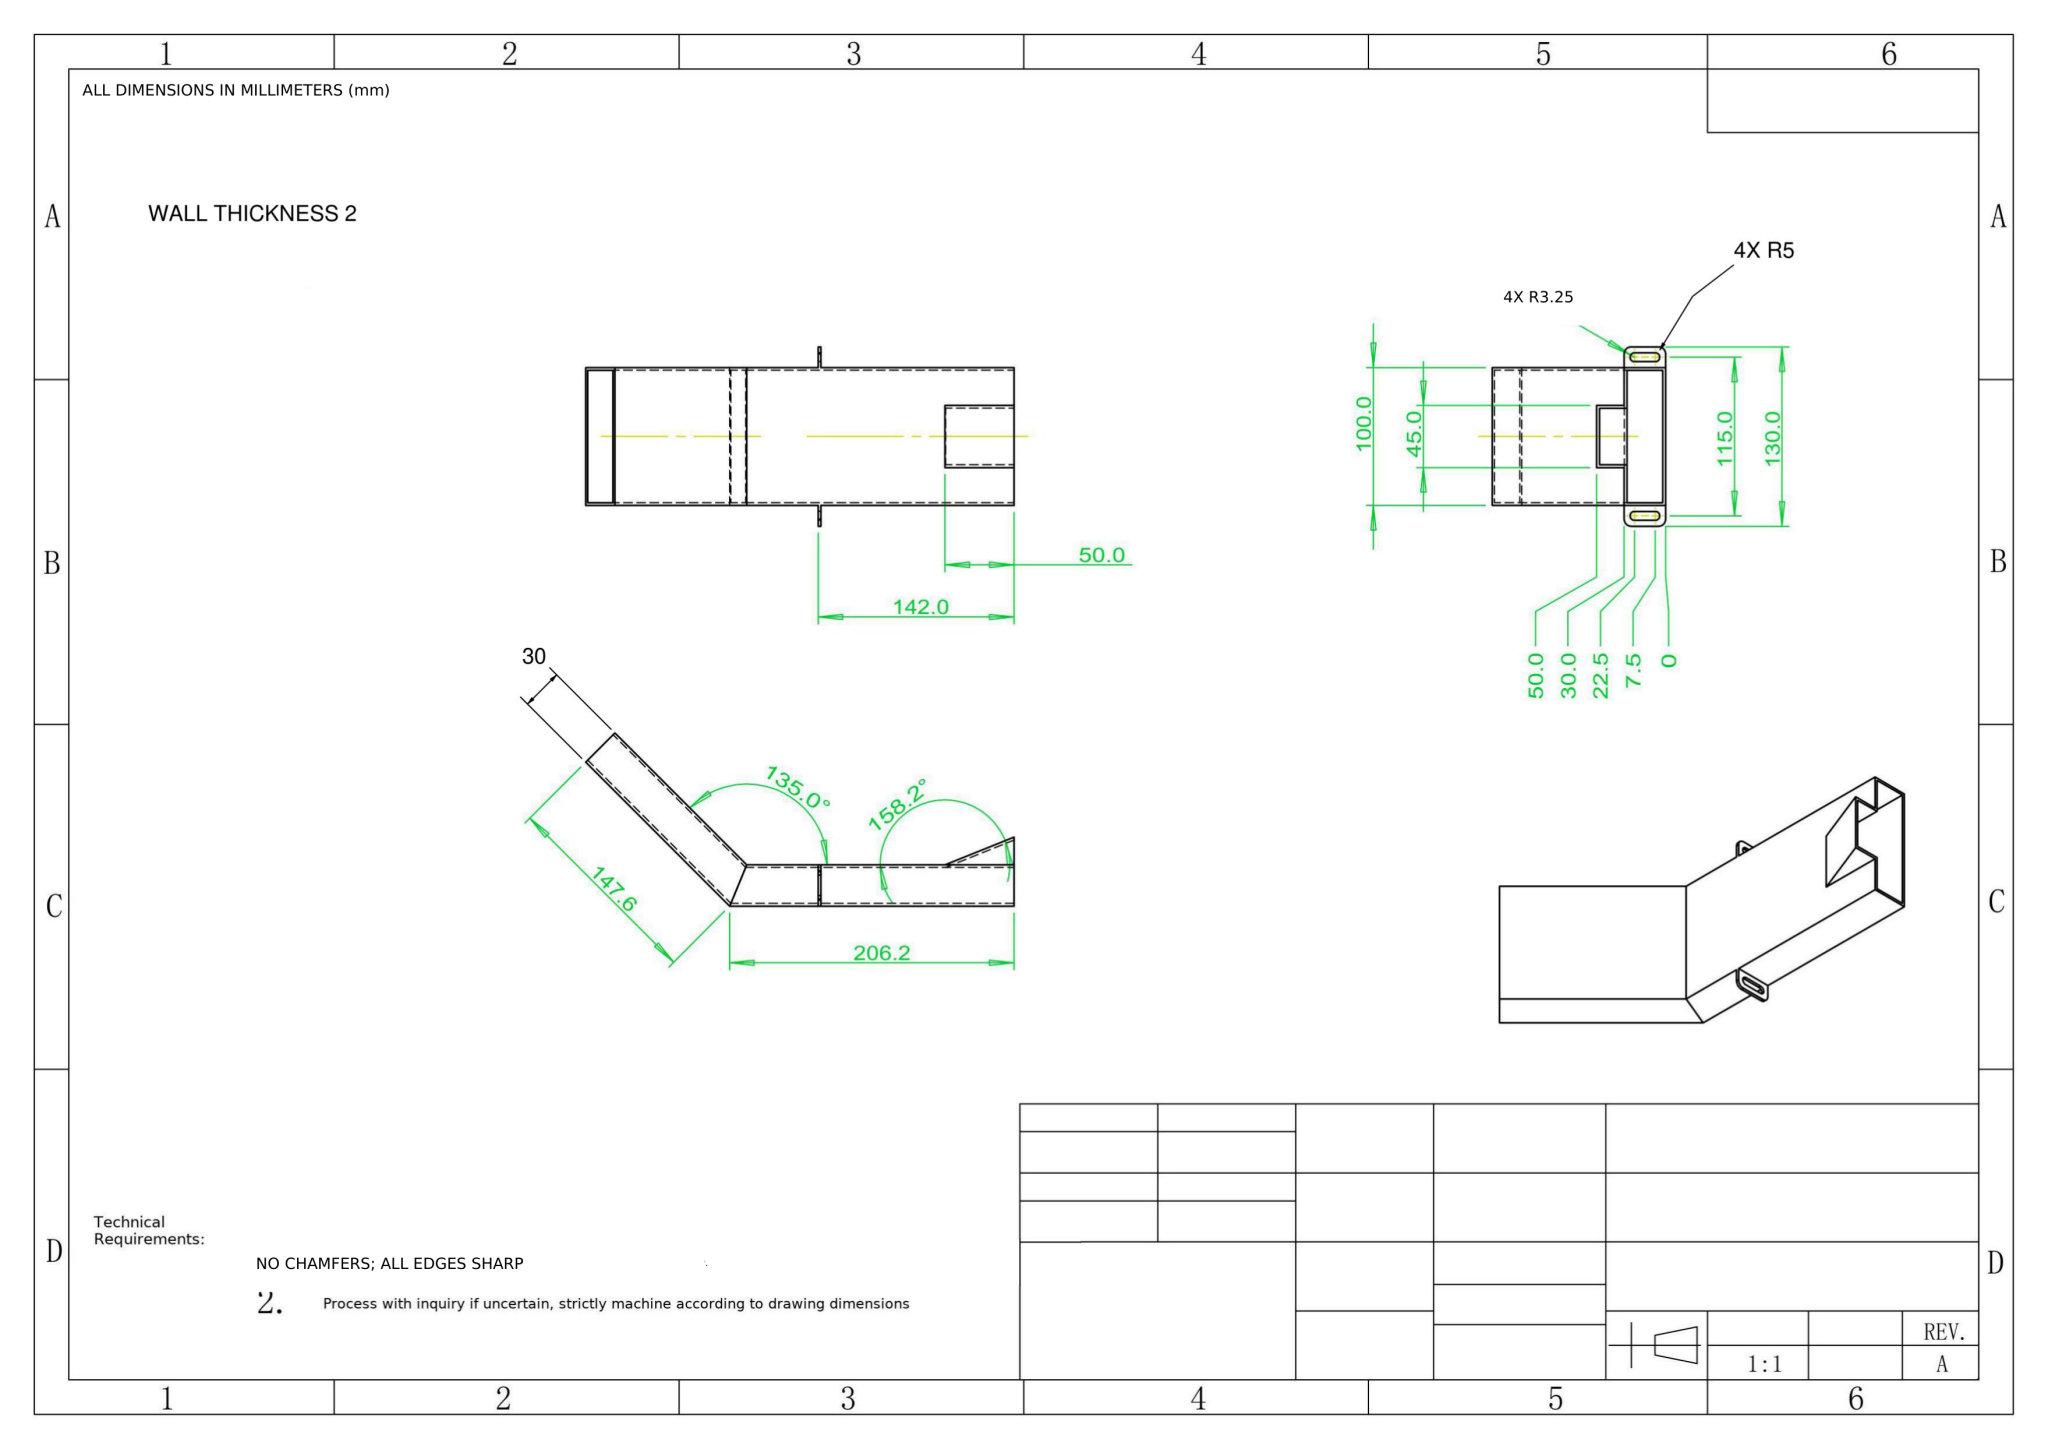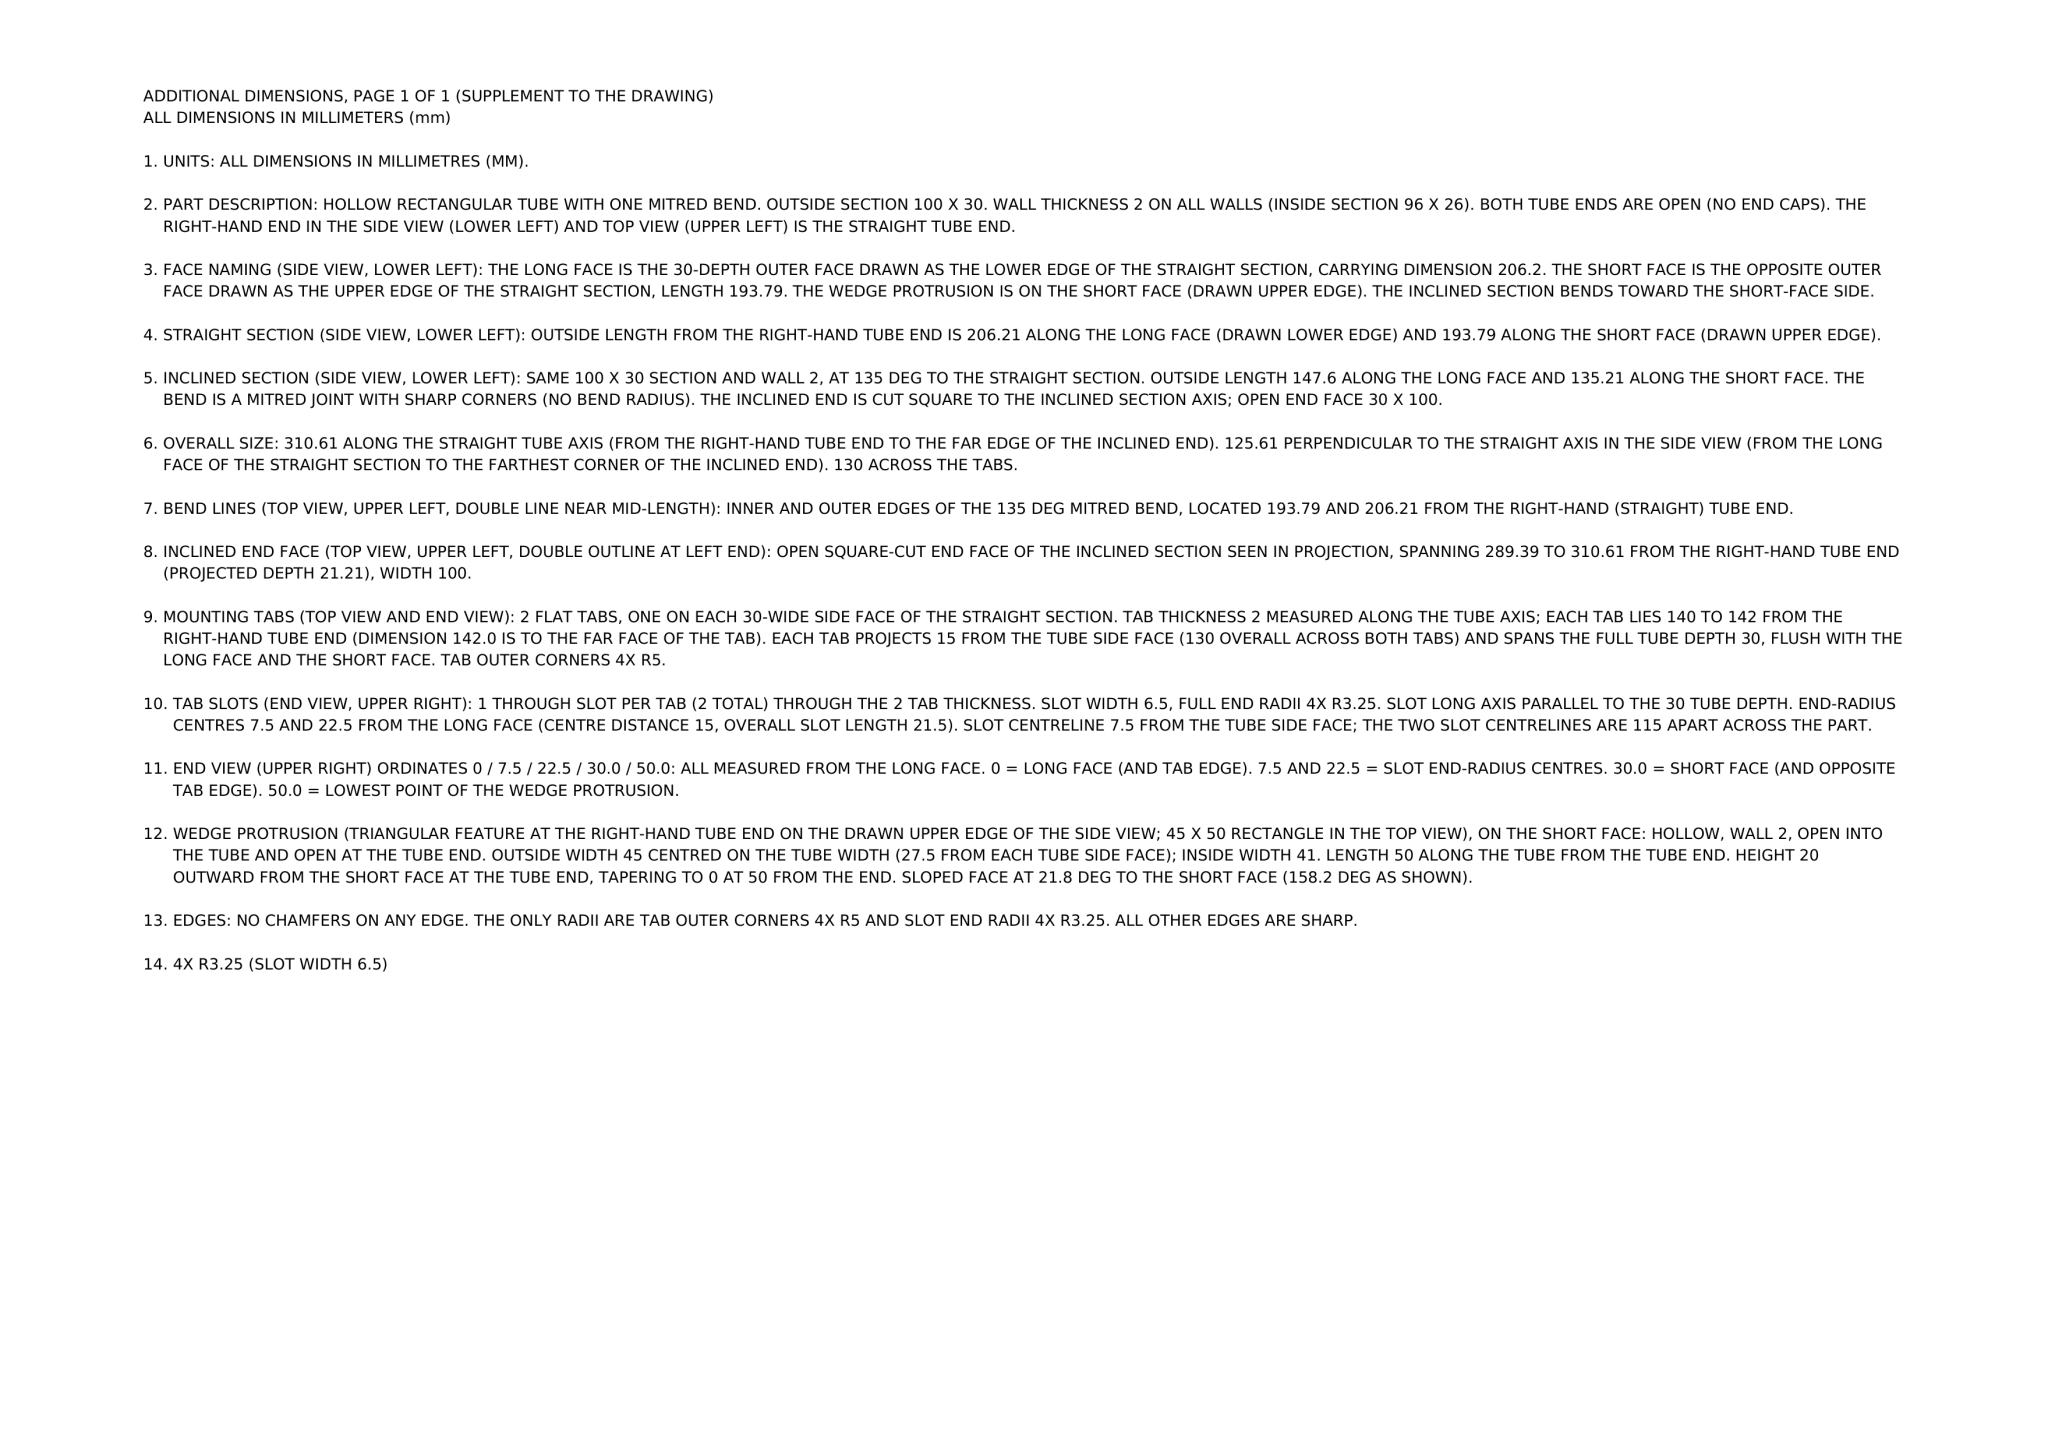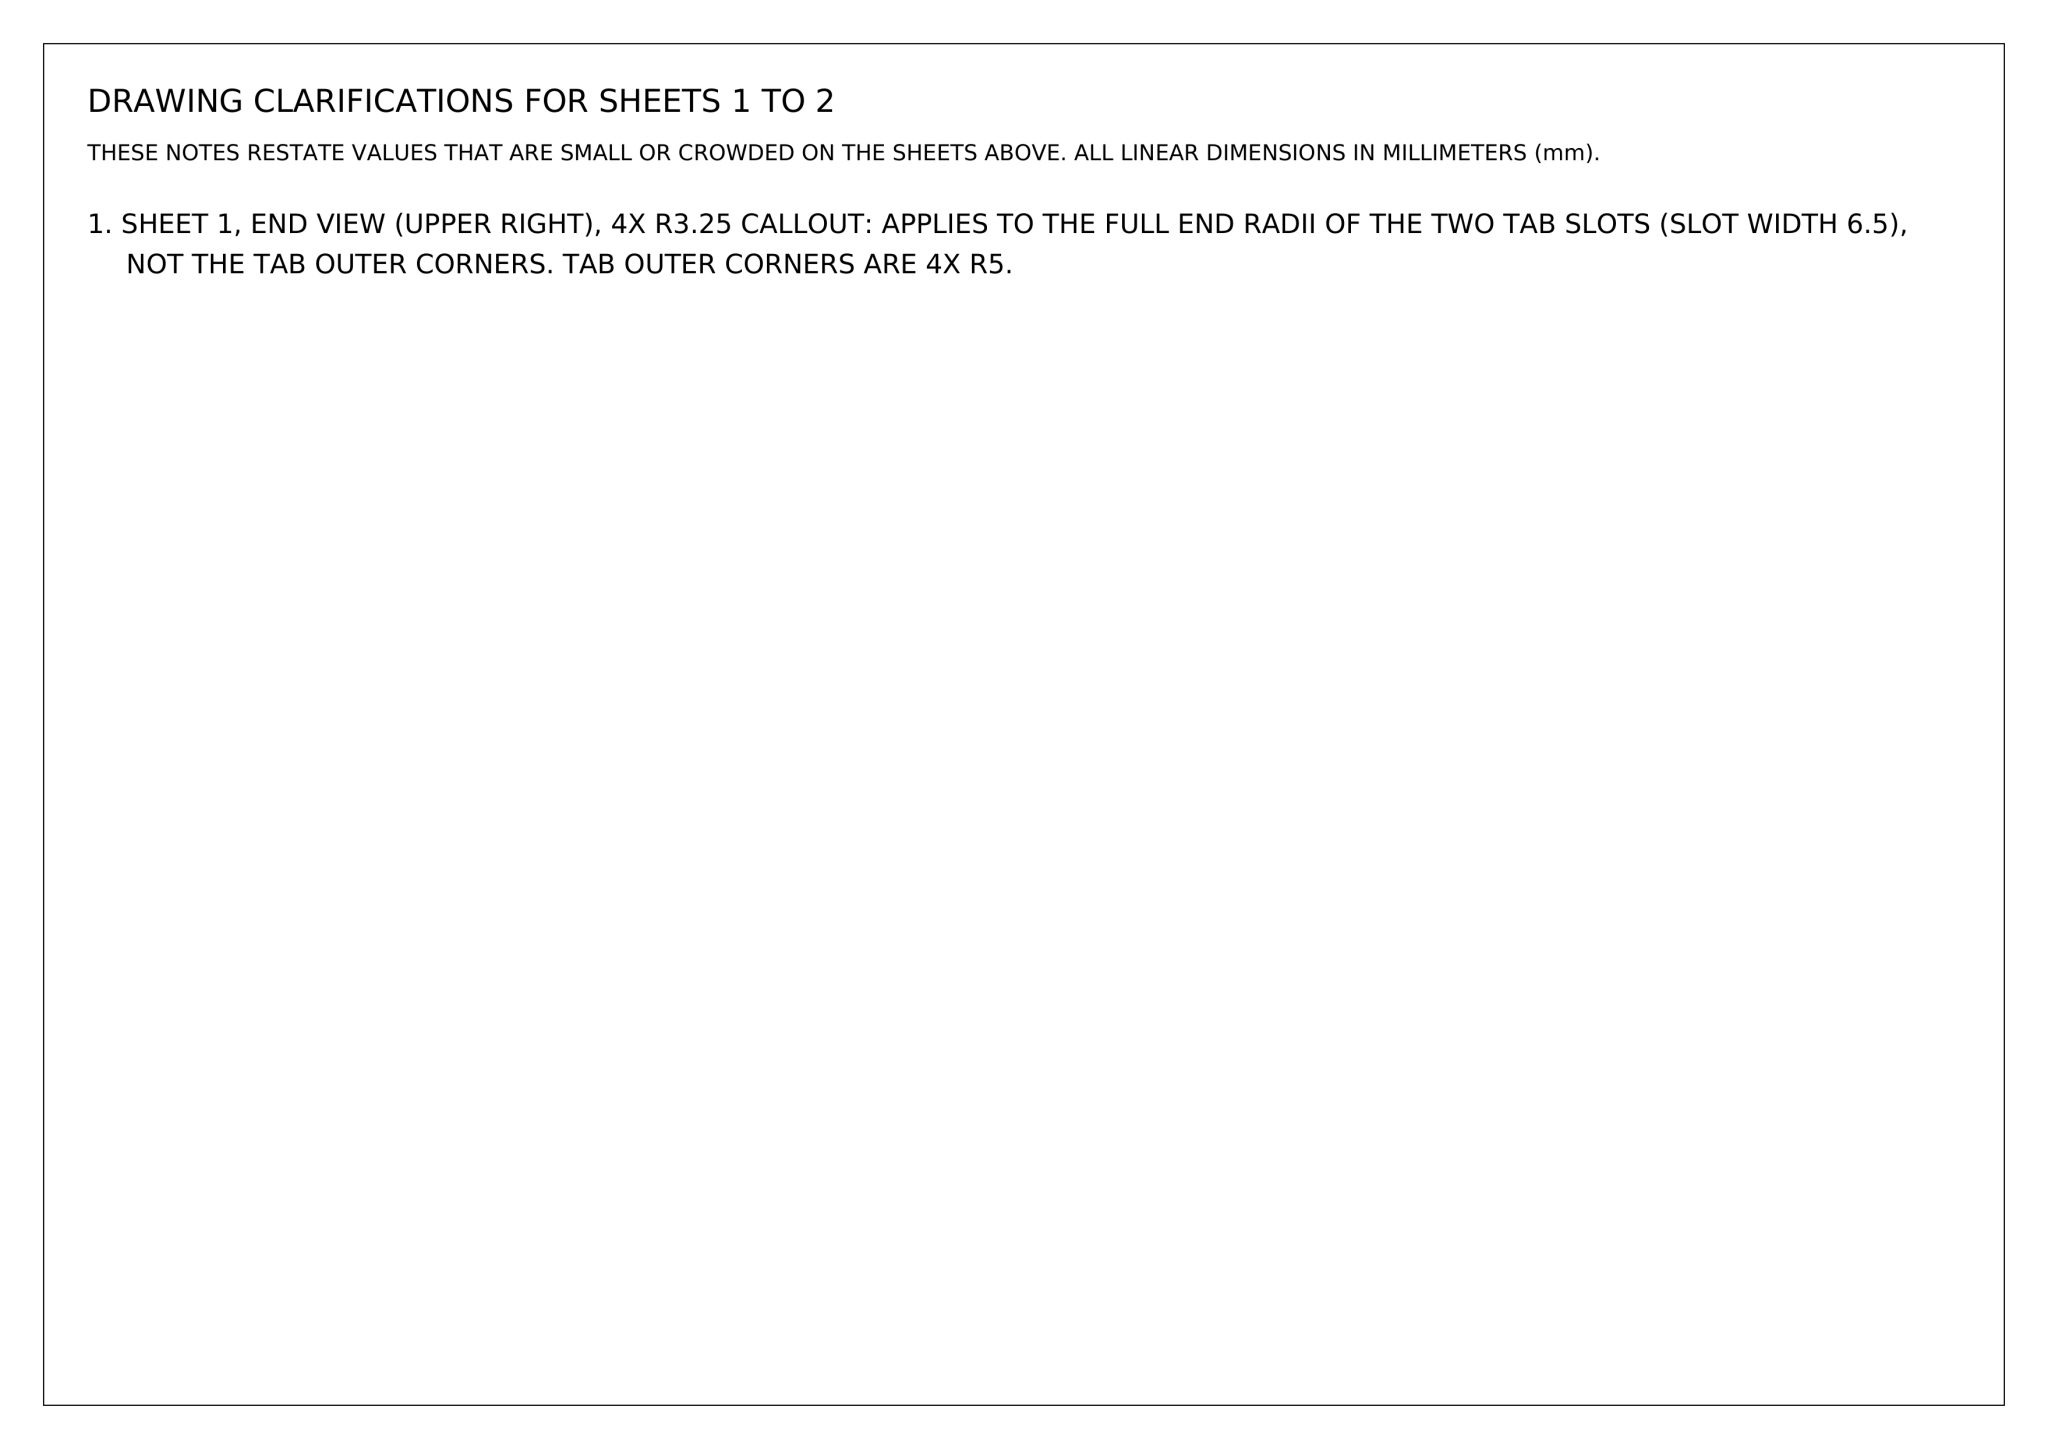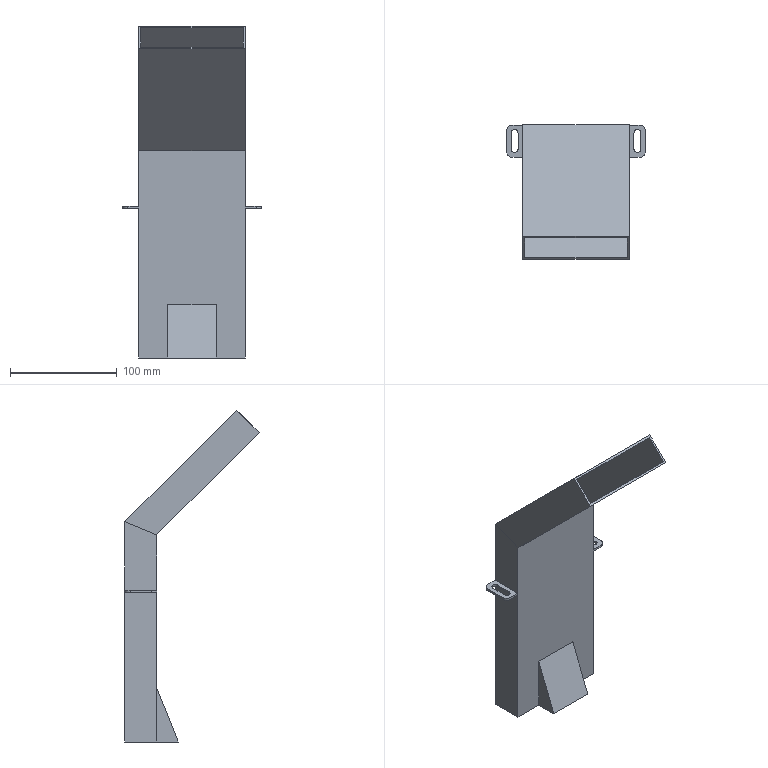Part | NX | mm | 1 solid | 46 faces | box 130 x 125.61 x 310.61 mm | volume 175625 mm3 | plane 36 | cylinder 10 | commonest cylinder face diameters 6.5 x6 10 x4